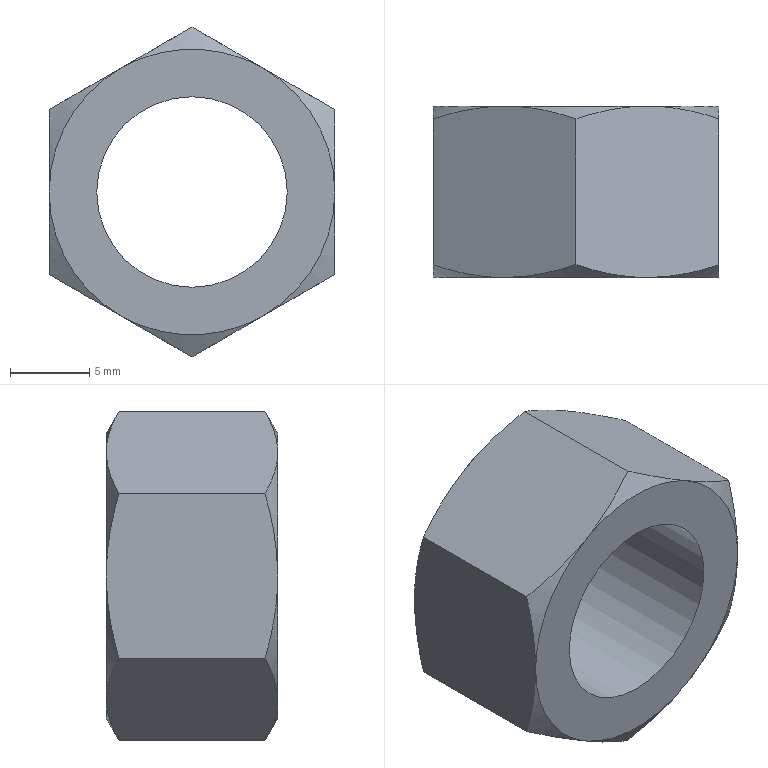Component | SolidWorks | GB_T6170-2000[Type1HexNutGradeAAndBM12]-1 | 1 solid | 22 faces | box 18 x 10.8 x 20.78 mm | volume 1796 mm3 | cone 12 | plane 8 | cylinder 2 | commonest cylinder face diameters 12 x2
build123d program:
from build123d import *

# Parameters (mm, degrees)
SKETCH1_R          = 6
BASE_EXTRUDE_DEPTH = 10.8
SKETCH2_OUTSIDE_W  = 89.934
SKETCH2_OUTSIDE_H  = 92.718
SKETCH2_OUTSIDE_R  = 9
CUT_EXTRUDE1_DEPTH = 18.483
CUT_EXTRUDE1_DRAFT = -60
SKETCH3_OUTSIDE_W  = 89.934
SKETCH3_OUTSIDE_H  = 92.718
SKETCH3_OUTSIDE_R  = 9
CUT_EXTRUDE2_DEPTH = 18.483
CUT_EXTRUDE2_DRAFT = -60


with BuildPart() as part:
    # Sketch1 → Base-Extrude (new body)
    with BuildSketch(Plane.XY):
        Polygon((0, 10.392), (-9, 5.196), (-9, -5.196), (0, -10.392), (9, -5.196), (9, 5.196), align=None)
        with Locations(Location((0, 0, 0), (0, 0, 180))):
            Circle(SKETCH1_R, mode=Mode.SUBTRACT)
    extrude(amount=BASE_EXTRUDE_DEPTH)


with BuildPart() as cut_extrude1_tool:
    # Sketch2 outside → Cut-Extrude1 (with draft: the straight prism first)
    with BuildSketch(Plane(origin=(0, 0, 0), x_dir=(-1, 0, 0), z_dir=(0, 0, -1))):
        Rectangle(SKETCH2_OUTSIDE_W, SKETCH2_OUTSIDE_H)
        Circle(SKETCH2_OUTSIDE_R, mode=Mode.SUBTRACT)
    extrude(amount=-CUT_EXTRUDE1_DEPTH)
    # Cut-Extrude1: the draft: its side faces are tilted about the plane it starts from
    cut_extrude1_sides = [cut_extrude1_tool.faces().sort_by_distance(p)[0] for p in [
        (0, -46.359, 9.241),
        (-44.967, 0, 9.241),
        (0, 46.359, 9.241),
        (44.967, 0, 9.241),
        (9, 0, 9.241),
    ]]
    draft(cut_extrude1_sides, Plane(origin=(0, 0, 0), x_dir=(-1, 0, 0), z_dir=(0, 0, -1)), CUT_EXTRUDE1_DRAFT)


with BuildPart() as part_1:
    add(part.part)

    # Cut-Extrude1: cut by cut_extrude1_tool
    add(cut_extrude1_tool.part, mode=Mode.SUBTRACT)


with BuildPart() as cut_extrude2_tool:
    # Sketch3 outside → Cut-Extrude2 (with draft: the straight prism first)
    with BuildSketch(Plane.XY.offset(10.8)):
        Rectangle(SKETCH3_OUTSIDE_W, SKETCH3_OUTSIDE_H)
        Circle(SKETCH3_OUTSIDE_R, mode=Mode.SUBTRACT)
    extrude(amount=-CUT_EXTRUDE2_DEPTH)
    # Cut-Extrude2: the draft: its side faces are tilted about the plane it starts from
    cut_extrude2_sides = [cut_extrude2_tool.faces().sort_by_distance(p)[0] for p in [
        (0, -46.359, 1.559),
        (44.967, 0, 1.559),
        (0, 46.359, 1.559),
        (-44.967, 0, 1.559),
        (-9, 0, 1.559),
    ]]
    draft(cut_extrude2_sides, Plane.XY.offset(10.8), CUT_EXTRUDE2_DRAFT)


with BuildPart() as part_2:
    add(part_1.part)

    # Cut-Extrude2: cut by cut_extrude2_tool
    add(cut_extrude2_tool.part, mode=Mode.SUBTRACT)


solid = part_2.part

# Placed as in the assembly
solid = solid.moved(Location((-380, -35.6, 90), (90, 0, 0)))
STEP:
#1=CARTESIAN_POINT('',(-15.197,-1.827,3.543));
#2=VERTEX_POINT('',#1);
#3=CARTESIAN_POINT('',(-14.724,-1.827,3.543));
#4=VERTEX_POINT('',#3);
#5=CARTESIAN_POINT('',(-14.961,-1.827,3.543));
#6=DIRECTION('',(0.,-1.,-0.));
#7=DIRECTION('',(1.,0.,0.));
#8=AXIS2_PLACEMENT_3D('',#5,#6,#7);
#9=CIRCLE('',#8,0.2362);
#10=EDGE_CURVE('',#2,#4,#9,.T.);
#11=ORIENTED_EDGE('',*,*,#10,.T.);
#12=CARTESIAN_POINT('',(-14.724,-1.402,3.543));
#13=VERTEX_POINT('',#12);
#14=CARTESIAN_POINT('',(-14.724,-1.827,3.543));
#15=DIRECTION('',(0.,1.,0.));
#16=VECTOR('',#15,39.37);
#17=LINE('',#14,#16);
#18=EDGE_CURVE('',#4,#13,#17,.T.);
#19=ORIENTED_EDGE('',*,*,#18,.T.);
#20=CARTESIAN_POINT('',(-15.197,-1.402,3.543));
#21=VERTEX_POINT('',#20);
#22=CARTESIAN_POINT('',(-14.961,-1.402,3.543));
#23=DIRECTION('',(0.,-1.,-0.));
#24=DIRECTION('',(1.,0.,0.));
#25=AXIS2_PLACEMENT_3D('',#22,#23,#24);
#26=CIRCLE('',#25,0.2362);
#27=EDGE_CURVE('',#21,#13,#26,.T.);
#28=ORIENTED_EDGE('',*,*,#27,.F.);
#29=CARTESIAN_POINT('',(-15.197,-1.827,3.543));
#30=DIRECTION('',(0.,1.,0.));
#31=VECTOR('',#30,39.37);
#32=LINE('',#29,#31);
#33=EDGE_CURVE('',#2,#21,#32,.T.);
#34=ORIENTED_EDGE('',*,*,#33,.F.);
#35=EDGE_LOOP('',(#11,#19,#28,#34));
#36=FACE_OUTER_BOUND('',#35,.T.);
#37=CARTESIAN_POINT('',(-14.961,-1.827,3.543));
#38=DIRECTION('',(0.,1.,0.));
#39=DIRECTION('',(-1.,0.,0.));
#40=AXIS2_PLACEMENT_3D('',#37,#38,#39);
#41=CYLINDRICAL_SURFACE('',#40,0.2362);
#42=ADVANCED_FACE('',(#36),#41,.F.);
#43=CARTESIAN_POINT('',(-14.606,-1.795,3.748));
#44=VERTEX_POINT('',#43);
#45=CARTESIAN_POINT('',(-14.783,-1.827,3.85));
#46=VERTEX_POINT('',#45);
#47=CARTESIAN_POINT('',(-14.606,-1.795,3.748));
#48=CARTESIAN_POINT('',(-14.635,-1.805,3.765));
#49=CARTESIAN_POINT('',(-14.664,-1.813,3.781));
#50=CARTESIAN_POINT('',(-14.723,-1.824,3.816));
#51=CARTESIAN_POINT('',(-14.753,-1.827,3.833));
#52=CARTESIAN_POINT('',(-14.783,-1.827,3.85));
#53=B_SPLINE_CURVE_WITH_KNOTS('',3,(#47,#48,#49,#50,#51,#52),.UNSPECIFIED.,.F.,.F.,(4,2,4),(0.00000024,0.002629,0.005258),.UNSPECIFIED.);
#54=EDGE_CURVE('',#44,#46,#53,.T.);
#55=ORIENTED_EDGE('',*,*,#54,.F.);
#56=CARTESIAN_POINT('',(-14.606,-1.433,3.748));
#57=VERTEX_POINT('',#56);
#58=CARTESIAN_POINT('',(-14.606,-1.827,3.748));
#59=DIRECTION('',(0.,1.,0.));
#60=VECTOR('',#59,39.37);
#61=LINE('',#58,#60);
#62=EDGE_CURVE('',#44,#57,#61,.T.);
#63=ORIENTED_EDGE('',*,*,#62,.T.);
#64=CARTESIAN_POINT('',(-14.783,-1.402,3.85));
#65=VERTEX_POINT('',#64);
#66=CARTESIAN_POINT('',(-14.783,-1.402,3.85));
#67=CARTESIAN_POINT('',(-14.768,-1.402,3.841));
#68=CARTESIAN_POINT('',(-14.753,-1.402,3.833));
#69=CARTESIAN_POINT('',(-14.723,-1.405,3.816));
#70=CARTESIAN_POINT('',(-14.709,-1.407,3.807));
#71=CARTESIAN_POINT('',(-14.664,-1.416,3.781));
#72=CARTESIAN_POINT('',(-14.635,-1.424,3.765));
#73=CARTESIAN_POINT('',(-14.606,-1.433,3.748));
#74=B_SPLINE_CURVE_WITH_KNOTS('',3,(#66,#67,#68,#69,#70,#71,#72,#73),.UNSPECIFIED.,.F.,.F.,(4,2,2,4),(0.005258,0.006567,0.007877,0.0105),.UNSPECIFIED.);
#75=EDGE_CURVE('',#65,#57,#74,.T.);
#76=ORIENTED_EDGE('',*,*,#75,.F.);
#77=CARTESIAN_POINT('',(-14.961,-1.433,3.952));
#78=VERTEX_POINT('',#77);
#79=CARTESIAN_POINT('',(-14.961,-1.433,3.952));
#80=CARTESIAN_POINT('',(-14.932,-1.424,3.936));
#81=CARTESIAN_POINT('',(-14.902,-1.416,3.919));
#82=CARTESIAN_POINT('',(-14.843,-1.405,3.885));
#83=CARTESIAN_POINT('',(-14.814,-1.402,3.868));
#84=CARTESIAN_POINT('',(-14.783,-1.402,3.85));
#85=B_SPLINE_CURVE_WITH_KNOTS('',3,(#79,#80,#81,#82,#83,#84),.UNSPECIFIED.,.F.,.F.,(4,2,4),(0.00000024,0.002629,0.005258),.UNSPECIFIED.);
#86=EDGE_CURVE('',#78,#65,#85,.T.);
#87=ORIENTED_EDGE('',*,*,#86,.F.);
#88=CARTESIAN_POINT('',(-14.961,-1.795,3.952));
#89=VERTEX_POINT('',#88);
#90=CARTESIAN_POINT('',(-14.961,-1.827,3.952));
#91=DIRECTION('',(0.,1.,0.));
#92=VECTOR('',#91,39.37);
#93=LINE('',#90,#92);
#94=EDGE_CURVE('',#89,#78,#93,.T.);
#95=ORIENTED_EDGE('',*,*,#94,.F.);
#96=CARTESIAN_POINT('',(-14.783,-1.827,3.85));
#97=CARTESIAN_POINT('',(-14.799,-1.827,3.859));
#98=CARTESIAN_POINT('',(-14.814,-1.826,3.868));
#99=CARTESIAN_POINT('',(-14.843,-1.823,3.885));
#100=CARTESIAN_POINT('',(-14.858,-1.821,3.893));
#101=CARTESIAN_POINT('',(-14.903,-1.813,3.919));
#102=CARTESIAN_POINT('',(-14.932,-1.805,3.936));
#103=CARTESIAN_POINT('',(-14.961,-1.795,3.952));
#104=B_SPLINE_CURVE_WITH_KNOTS('',3,(#96,#97,#98,#99,#100,#101,#102,#103),.UNSPECIFIED.,.F.,.F.,(4,2,2,4),(0.005258,0.006567,0.007877,0.0105),.UNSPECIFIED.);
#105=EDGE_CURVE('',#46,#89,#104,.T.);
#106=ORIENTED_EDGE('',*,*,#105,.F.);
#107=EDGE_LOOP('',(#55,#63,#76,#87,#95,#106));
#108=FACE_OUTER_BOUND('',#107,.T.);
#109=CARTESIAN_POINT('',(-14.606,-1.827,3.748));
#110=DIRECTION('',(-0.5,0.,-0.866));
#111=DIRECTION('',(0.866,0.,-0.5));
#112=AXIS2_PLACEMENT_3D('',#109,#110,#111);
#113=PLANE('',#112);
#114=ADVANCED_FACE('',(#108),#113,.F.);
#115=CARTESIAN_POINT('',(-15.138,-1.827,3.85));
#116=VERTEX_POINT('',#115);
#117=CARTESIAN_POINT('',(-14.961,-1.795,3.952));
#118=CARTESIAN_POINT('',(-14.99,-1.805,3.936));
#119=CARTESIAN_POINT('',(-15.019,-1.813,3.919));
#120=CARTESIAN_POINT('',(-15.078,-1.824,3.885));
#121=CARTESIAN_POINT('',(-15.108,-1.827,3.868));
#122=CARTESIAN_POINT('',(-15.138,-1.827,3.85));
#123=B_SPLINE_CURVE_WITH_KNOTS('',3,(#117,#118,#119,#120,#121,#122),.UNSPECIFIED.,.F.,.F.,(4,2,4),(0.00000024,0.002629,0.005258),.UNSPECIFIED.);
#124=EDGE_CURVE('',#89,#116,#123,.T.);
#125=ORIENTED_EDGE('',*,*,#124,.F.);
#126=ORIENTED_EDGE('',*,*,#94,.T.);
#127=CARTESIAN_POINT('',(-15.138,-1.402,3.85));
#128=VERTEX_POINT('',#127);
#129=CARTESIAN_POINT('',(-15.138,-1.402,3.85));
#130=CARTESIAN_POINT('',(-15.123,-1.402,3.859));
#131=CARTESIAN_POINT('',(-15.108,-1.402,3.868));
#132=CARTESIAN_POINT('',(-15.078,-1.405,3.885));
#133=CARTESIAN_POINT('',(-15.063,-1.407,3.893));
#134=CARTESIAN_POINT('',(-15.019,-1.416,3.919));
#135=CARTESIAN_POINT('',(-14.99,-1.424,3.936));
#136=CARTESIAN_POINT('',(-14.961,-1.433,3.952));
#137=B_SPLINE_CURVE_WITH_KNOTS('',3,(#129,#130,#131,#132,#133,#134,#135,#136),.UNSPECIFIED.,.F.,.F.,(4,2,2,4),(0.005258,0.006567,0.007877,0.0105),.UNSPECIFIED.);
#138=EDGE_CURVE('',#128,#78,#137,.T.);
#139=ORIENTED_EDGE('',*,*,#138,.F.);
#140=CARTESIAN_POINT('',(-15.315,-1.433,3.748));
#141=VERTEX_POINT('',#140);
#142=CARTESIAN_POINT('',(-15.315,-1.433,3.748));
#143=CARTESIAN_POINT('',(-15.286,-1.424,3.765));
#144=CARTESIAN_POINT('',(-15.257,-1.416,3.781));
#145=CARTESIAN_POINT('',(-15.198,-1.405,3.816));
#146=CARTESIAN_POINT('',(-15.168,-1.402,3.833));
#147=CARTESIAN_POINT('',(-15.138,-1.402,3.85));
#148=B_SPLINE_CURVE_WITH_KNOTS('',3,(#142,#143,#144,#145,#146,#147),.UNSPECIFIED.,.F.,.F.,(4,2,4),(0.00000024,0.002629,0.005258),.UNSPECIFIED.);
#149=EDGE_CURVE('',#141,#128,#148,.T.);
#150=ORIENTED_EDGE('',*,*,#149,.F.);
#151=CARTESIAN_POINT('',(-15.315,-1.795,3.748));
#152=VERTEX_POINT('',#151);
#153=CARTESIAN_POINT('',(-15.315,-1.827,3.748));
#154=DIRECTION('',(0.,1.,0.));
#155=VECTOR('',#154,39.37);
#156=LINE('',#153,#155);
#157=EDGE_CURVE('',#152,#141,#156,.T.);
#158=ORIENTED_EDGE('',*,*,#157,.F.);
#159=CARTESIAN_POINT('',(-15.138,-1.827,3.85));
#160=CARTESIAN_POINT('',(-15.153,-1.827,3.841));
#161=CARTESIAN_POINT('',(-15.168,-1.826,3.833));
#162=CARTESIAN_POINT('',(-15.198,-1.823,3.816));
#163=CARTESIAN_POINT('',(-15.213,-1.821,3.807));
#164=CARTESIAN_POINT('',(-15.257,-1.813,3.781));
#165=CARTESIAN_POINT('',(-15.286,-1.805,3.765));
#166=CARTESIAN_POINT('',(-15.315,-1.795,3.748));
#167=B_SPLINE_CURVE_WITH_KNOTS('',3,(#159,#160,#161,#162,#163,#164,#165,#166),.UNSPECIFIED.,.F.,.F.,(4,2,2,4),(0.005258,0.006567,0.007877,0.0105),.UNSPECIFIED.);
#168=EDGE_CURVE('',#116,#152,#167,.T.);
#169=ORIENTED_EDGE('',*,*,#168,.F.);
#170=EDGE_LOOP('',(#125,#126,#139,#150,#158,#169));
#171=FACE_OUTER_BOUND('',#170,.T.);
#172=CARTESIAN_POINT('',(-14.961,-1.827,3.952));
#173=DIRECTION('',(0.5,0.,-0.866));
#174=DIRECTION('',(0.866,-0.,0.5));
#175=AXIS2_PLACEMENT_3D('',#172,#173,#174);
#176=PLANE('',#175);
#177=ADVANCED_FACE('',(#171),#176,.F.);
#178=CARTESIAN_POINT('',(-15.315,-1.827,3.543));
#179=VERTEX_POINT('',#178);
#180=CARTESIAN_POINT('',(-15.315,-1.795,3.748));
#181=CARTESIAN_POINT('',(-15.315,-1.805,3.715));
#182=CARTESIAN_POINT('',(-15.315,-1.813,3.681));
#183=CARTESIAN_POINT('',(-15.315,-1.821,3.63));
#184=CARTESIAN_POINT('',(-15.315,-1.823,3.613));
#185=CARTESIAN_POINT('',(-15.315,-1.826,3.578));
#186=CARTESIAN_POINT('',(-15.315,-1.827,3.561));
#187=CARTESIAN_POINT('',(-15.315,-1.827,3.543));
#188=B_SPLINE_CURVE_WITH_KNOTS('',3,(#180,#181,#182,#183,#184,#185,#186,#187),.UNSPECIFIED.,.F.,.F.,(4,2,2,4),(0.02958,0.03221,0.03352,0.03484),.UNSPECIFIED.);
#189=EDGE_CURVE('',#152,#179,#188,.T.);
#190=ORIENTED_EDGE('',*,*,#189,.F.);
#191=ORIENTED_EDGE('',*,*,#157,.T.);
#192=CARTESIAN_POINT('',(-15.315,-1.402,3.543));
#193=VERTEX_POINT('',#192);
#194=CARTESIAN_POINT('',(-15.315,-1.402,3.543));
#195=CARTESIAN_POINT('',(-15.315,-1.402,3.561));
#196=CARTESIAN_POINT('',(-15.315,-1.402,3.578));
#197=CARTESIAN_POINT('',(-15.315,-1.405,3.613));
#198=CARTESIAN_POINT('',(-15.315,-1.407,3.63));
#199=CARTESIAN_POINT('',(-15.315,-1.416,3.681));
#200=CARTESIAN_POINT('',(-15.315,-1.424,3.715));
#201=CARTESIAN_POINT('',(-15.315,-1.433,3.748));
#202=B_SPLINE_CURVE_WITH_KNOTS('',3,(#194,#195,#196,#197,#198,#199,#200,#201),.UNSPECIFIED.,.F.,.F.,(4,2,2,4),(0.01478,0.01609,0.01741,0.02004),.UNSPECIFIED.);
#203=EDGE_CURVE('',#193,#141,#202,.T.);
#204=ORIENTED_EDGE('',*,*,#203,.F.);
#205=CARTESIAN_POINT('',(-15.315,-1.433,3.339));
#206=VERTEX_POINT('',#205);
#207=CARTESIAN_POINT('',(-15.315,-1.433,3.339));
#208=CARTESIAN_POINT('',(-15.315,-1.424,3.372));
#209=CARTESIAN_POINT('',(-15.315,-1.416,3.406));
#210=CARTESIAN_POINT('',(-15.315,-1.405,3.474));
#211=CARTESIAN_POINT('',(-15.315,-1.402,3.509));
#212=CARTESIAN_POINT('',(-15.315,-1.402,3.543));
#213=B_SPLINE_CURVE_WITH_KNOTS('',3,(#207,#208,#209,#210,#211,#212),.UNSPECIFIED.,.F.,.F.,(4,2,4),(0.009518,0.01215,0.01478),.UNSPECIFIED.);
#214=EDGE_CURVE('',#206,#193,#213,.T.);
#215=ORIENTED_EDGE('',*,*,#214,.F.);
#216=CARTESIAN_POINT('',(-15.315,-1.795,3.339));
#217=VERTEX_POINT('',#216);
#218=CARTESIAN_POINT('',(-15.315,-1.827,3.339));
#219=DIRECTION('',(0.,1.,0.));
#220=VECTOR('',#219,39.37);
#221=LINE('',#218,#220);
#222=EDGE_CURVE('',#217,#206,#221,.T.);
#223=ORIENTED_EDGE('',*,*,#222,.F.);
#224=CARTESIAN_POINT('',(-15.315,-1.827,3.543));
#225=CARTESIAN_POINT('',(-15.315,-1.827,3.509));
#226=CARTESIAN_POINT('',(-15.315,-1.824,3.474));
#227=CARTESIAN_POINT('',(-15.315,-1.813,3.406));
#228=CARTESIAN_POINT('',(-15.315,-1.805,3.372));
#229=CARTESIAN_POINT('',(-15.315,-1.795,3.339));
#230=B_SPLINE_CURVE_WITH_KNOTS('',3,(#224,#225,#226,#227,#228,#229),.UNSPECIFIED.,.F.,.F.,(4,2,4),(0.03484,0.03747,0.0401),.UNSPECIFIED.);
#231=EDGE_CURVE('',#179,#217,#230,.T.);
#232=ORIENTED_EDGE('',*,*,#231,.F.);
#233=EDGE_LOOP('',(#190,#191,#204,#215,#223,#232));
#234=FACE_OUTER_BOUND('',#233,.T.);
#235=CARTESIAN_POINT('',(-15.315,-1.827,3.748));
#236=DIRECTION('',(1.,-0.,0.));
#237=DIRECTION('',(-0.,-0.,1.));
#238=AXIS2_PLACEMENT_3D('',#235,#236,#237);
#239=PLANE('',#238);
#240=ADVANCED_FACE('',(#234),#239,.F.);
#241=CARTESIAN_POINT('',(-15.138,-1.827,3.236));
#242=VERTEX_POINT('',#241);
#243=CARTESIAN_POINT('',(-15.315,-1.795,3.339));
#244=CARTESIAN_POINT('',(-15.286,-1.805,3.322));
#245=CARTESIAN_POINT('',(-15.257,-1.813,3.305));
#246=CARTESIAN_POINT('',(-15.198,-1.824,3.271));
#247=CARTESIAN_POINT('',(-15.168,-1.827,3.254));
#248=CARTESIAN_POINT('',(-15.138,-1.827,3.236));
#249=B_SPLINE_CURVE_WITH_KNOTS('',3,(#243,#244,#245,#246,#247,#248),.UNSPECIFIED.,.F.,.F.,(4,2,4),(0.00000024,0.002629,0.005258),.UNSPECIFIED.);
#250=EDGE_CURVE('',#217,#242,#249,.T.);
#251=ORIENTED_EDGE('',*,*,#250,.F.);
#252=ORIENTED_EDGE('',*,*,#222,.T.);
#253=CARTESIAN_POINT('',(-15.138,-1.402,3.236));
#254=VERTEX_POINT('',#253);
#255=CARTESIAN_POINT('',(-15.138,-1.402,3.236));
#256=CARTESIAN_POINT('',(-15.153,-1.402,3.245));
#257=CARTESIAN_POINT('',(-15.168,-1.402,3.254));
#258=CARTESIAN_POINT('',(-15.198,-1.405,3.271));
#259=CARTESIAN_POINT('',(-15.213,-1.407,3.28));
#260=CARTESIAN_POINT('',(-15.257,-1.416,3.305));
#261=CARTESIAN_POINT('',(-15.286,-1.424,3.322));
#262=CARTESIAN_POINT('',(-15.315,-1.433,3.339));
#263=B_SPLINE_CURVE_WITH_KNOTS('',3,(#255,#256,#257,#258,#259,#260,#261,#262),.UNSPECIFIED.,.F.,.F.,(4,2,2,4),(0.005258,0.006567,0.007877,0.0105),.UNSPECIFIED.);
#264=EDGE_CURVE('',#254,#206,#263,.T.);
#265=ORIENTED_EDGE('',*,*,#264,.F.);
#266=CARTESIAN_POINT('',(-14.961,-1.433,3.134));
#267=VERTEX_POINT('',#266);
#268=CARTESIAN_POINT('',(-14.961,-1.433,3.134));
#269=CARTESIAN_POINT('',(-14.99,-1.424,3.151));
#270=CARTESIAN_POINT('',(-15.019,-1.416,3.168));
#271=CARTESIAN_POINT('',(-15.078,-1.405,3.202));
#272=CARTESIAN_POINT('',(-15.108,-1.402,3.219));
#273=CARTESIAN_POINT('',(-15.138,-1.402,3.236));
#274=B_SPLINE_CURVE_WITH_KNOTS('',3,(#268,#269,#270,#271,#272,#273),.UNSPECIFIED.,.F.,.F.,(4,2,4),(0.00000024,0.002629,0.005258),.UNSPECIFIED.);
#275=EDGE_CURVE('',#267,#254,#274,.T.);
#276=ORIENTED_EDGE('',*,*,#275,.F.);
#277=CARTESIAN_POINT('',(-14.961,-1.795,3.134));
#278=VERTEX_POINT('',#277);
#279=CARTESIAN_POINT('',(-14.961,-1.827,3.134));
#280=DIRECTION('',(0.,1.,0.));
#281=VECTOR('',#280,39.37);
#282=LINE('',#279,#281);
#283=EDGE_CURVE('',#278,#267,#282,.T.);
#284=ORIENTED_EDGE('',*,*,#283,.F.);
#285=CARTESIAN_POINT('',(-15.138,-1.827,3.236));
#286=CARTESIAN_POINT('',(-15.123,-1.827,3.228));
#287=CARTESIAN_POINT('',(-15.108,-1.826,3.219));
#288=CARTESIAN_POINT('',(-15.078,-1.823,3.202));
#289=CARTESIAN_POINT('',(-15.063,-1.821,3.193));
#290=CARTESIAN_POINT('',(-15.019,-1.813,3.168));
#291=CARTESIAN_POINT('',(-14.99,-1.805,3.151));
#292=CARTESIAN_POINT('',(-14.961,-1.795,3.134));
#293=B_SPLINE_CURVE_WITH_KNOTS('',3,(#285,#286,#287,#288,#289,#290,#291,#292),.UNSPECIFIED.,.F.,.F.,(4,2,2,4),(0.005258,0.006567,0.007877,0.0105),.UNSPECIFIED.);
#294=EDGE_CURVE('',#242,#278,#293,.T.);
#295=ORIENTED_EDGE('',*,*,#294,.F.);
#296=EDGE_LOOP('',(#251,#252,#265,#276,#284,#295));
#297=FACE_OUTER_BOUND('',#296,.T.);
#298=CARTESIAN_POINT('',(-15.315,-1.827,3.339));
#299=DIRECTION('',(0.5,-0.,0.866));
#300=DIRECTION('',(-0.866,-0.,0.5));
#301=AXIS2_PLACEMENT_3D('',#298,#299,#300);
#302=PLANE('',#301);
#303=ADVANCED_FACE('',(#297),#302,.F.);
#304=CARTESIAN_POINT('',(-14.783,-1.827,3.236));
#305=VERTEX_POINT('',#304);
#306=CARTESIAN_POINT('',(-14.961,-1.795,3.134));
#307=CARTESIAN_POINT('',(-14.932,-1.805,3.151));
#308=CARTESIAN_POINT('',(-14.902,-1.813,3.168));
#309=CARTESIAN_POINT('',(-14.843,-1.824,3.202));
#310=CARTESIAN_POINT('',(-14.814,-1.827,3.219));
#311=CARTESIAN_POINT('',(-14.783,-1.827,3.236));
#312=B_SPLINE_CURVE_WITH_KNOTS('',3,(#306,#307,#308,#309,#310,#311),.UNSPECIFIED.,.F.,.F.,(4,2,4),(0.00000024,0.002629,0.005258),.UNSPECIFIED.);
#313=EDGE_CURVE('',#278,#305,#312,.T.);
#314=ORIENTED_EDGE('',*,*,#313,.F.);
#315=ORIENTED_EDGE('',*,*,#283,.T.);
#316=CARTESIAN_POINT('',(-14.783,-1.402,3.236));
#317=VERTEX_POINT('',#316);
#318=CARTESIAN_POINT('',(-14.783,-1.402,3.236));
#319=CARTESIAN_POINT('',(-14.799,-1.402,3.228));
#320=CARTESIAN_POINT('',(-14.814,-1.402,3.219));
#321=CARTESIAN_POINT('',(-14.843,-1.405,3.202));
#322=CARTESIAN_POINT('',(-14.858,-1.407,3.193));
#323=CARTESIAN_POINT('',(-14.903,-1.416,3.168));
#324=CARTESIAN_POINT('',(-14.932,-1.424,3.151));
#325=CARTESIAN_POINT('',(-14.961,-1.433,3.134));
#326=B_SPLINE_CURVE_WITH_KNOTS('',3,(#318,#319,#320,#321,#322,#323,#324,#325),.UNSPECIFIED.,.F.,.F.,(4,2,2,4),(0.005258,0.006567,0.007877,0.0105),.UNSPECIFIED.);
#327=EDGE_CURVE('',#317,#267,#326,.T.);
#328=ORIENTED_EDGE('',*,*,#327,.F.);
#329=CARTESIAN_POINT('',(-14.606,-1.433,3.339));
#330=VERTEX_POINT('',#329);
#331=CARTESIAN_POINT('',(-14.606,-1.433,3.339));
#332=CARTESIAN_POINT('',(-14.635,-1.424,3.322));
#333=CARTESIAN_POINT('',(-14.664,-1.416,3.305));
#334=CARTESIAN_POINT('',(-14.723,-1.405,3.271));
#335=CARTESIAN_POINT('',(-14.753,-1.402,3.254));
#336=CARTESIAN_POINT('',(-14.783,-1.402,3.236));
#337=B_SPLINE_CURVE_WITH_KNOTS('',3,(#331,#332,#333,#334,#335,#336),.UNSPECIFIED.,.F.,.F.,(4,2,4),(0.00000024,0.002629,0.005258),.UNSPECIFIED.);
#338=EDGE_CURVE('',#330,#317,#337,.T.);
#339=ORIENTED_EDGE('',*,*,#338,.F.);
#340=CARTESIAN_POINT('',(-14.606,-1.795,3.339));
#341=VERTEX_POINT('',#340);
#342=CARTESIAN_POINT('',(-14.606,-1.827,3.339));
#343=DIRECTION('',(0.,1.,0.));
#344=VECTOR('',#343,39.37);
#345=LINE('',#342,#344);
#346=EDGE_CURVE('',#341,#330,#345,.T.);
#347=ORIENTED_EDGE('',*,*,#346,.F.);
#348=CARTESIAN_POINT('',(-14.783,-1.827,3.236));
#349=CARTESIAN_POINT('',(-14.768,-1.827,3.245));
#350=CARTESIAN_POINT('',(-14.753,-1.826,3.254));
#351=CARTESIAN_POINT('',(-14.723,-1.823,3.271));
#352=CARTESIAN_POINT('',(-14.709,-1.821,3.28));
#353=CARTESIAN_POINT('',(-14.664,-1.813,3.305));
#354=CARTESIAN_POINT('',(-14.635,-1.805,3.322));
#355=CARTESIAN_POINT('',(-14.606,-1.795,3.339));
#356=B_SPLINE_CURVE_WITH_KNOTS('',3,(#348,#349,#350,#351,#352,#353,#354,#355),.UNSPECIFIED.,.F.,.F.,(4,2,2,4),(0.005258,0.006567,0.007877,0.0105),.UNSPECIFIED.);
#357=EDGE_CURVE('',#305,#341,#356,.T.);
#358=ORIENTED_EDGE('',*,*,#357,.F.);
#359=EDGE_LOOP('',(#314,#315,#328,#339,#347,#358));
#360=FACE_OUTER_BOUND('',#359,.T.);
#361=CARTESIAN_POINT('',(-14.961,-1.827,3.134));
#362=DIRECTION('',(-0.5,-0.,0.866));
#363=DIRECTION('',(-0.866,0.,-0.5));
#364=AXIS2_PLACEMENT_3D('',#361,#362,#363);
#365=PLANE('',#364);
#366=ADVANCED_FACE('',(#360),#365,.F.);
#367=CARTESIAN_POINT('',(-14.606,-1.827,3.543));
#368=VERTEX_POINT('',#367);
#369=CARTESIAN_POINT('',(-14.606,-1.795,3.339));
#370=CARTESIAN_POINT('',(-14.606,-1.805,3.372));
#371=CARTESIAN_POINT('',(-14.606,-1.813,3.406));
#372=CARTESIAN_POINT('',(-14.606,-1.824,3.474));
#373=CARTESIAN_POINT('',(-14.606,-1.827,3.509));
#374=CARTESIAN_POINT('',(-14.606,-1.827,3.543));
#375=B_SPLINE_CURVE_WITH_KNOTS('',3,(#369,#370,#371,#372,#373,#374),.UNSPECIFIED.,.F.,.F.,(4,2,4),(0.009518,0.01215,0.01478),.UNSPECIFIED.);
#376=EDGE_CURVE('',#341,#368,#375,.T.);
#377=ORIENTED_EDGE('',*,*,#376,.F.);
#378=ORIENTED_EDGE('',*,*,#346,.T.);
#379=CARTESIAN_POINT('',(-14.606,-1.402,3.543));
#380=VERTEX_POINT('',#379);
#381=CARTESIAN_POINT('',(-14.606,-1.402,3.543));
#382=CARTESIAN_POINT('',(-14.606,-1.402,3.509));
#383=CARTESIAN_POINT('',(-14.606,-1.405,3.474));
#384=CARTESIAN_POINT('',(-14.606,-1.416,3.406));
#385=CARTESIAN_POINT('',(-14.606,-1.424,3.372));
#386=CARTESIAN_POINT('',(-14.606,-1.433,3.339));
#387=B_SPLINE_CURVE_WITH_KNOTS('',3,(#381,#382,#383,#384,#385,#386),.UNSPECIFIED.,.F.,.F.,(4,2,4),(0.03484,0.03747,0.0401),.UNSPECIFIED.);
#388=EDGE_CURVE('',#380,#330,#387,.T.);
#389=ORIENTED_EDGE('',*,*,#388,.F.);
#390=CARTESIAN_POINT('',(-14.606,-1.433,3.748));
#391=CARTESIAN_POINT('',(-14.606,-1.424,3.715));
#392=CARTESIAN_POINT('',(-14.606,-1.416,3.681));
#393=CARTESIAN_POINT('',(-14.606,-1.407,3.63));
#394=CARTESIAN_POINT('',(-14.606,-1.405,3.613));
#395=CARTESIAN_POINT('',(-14.606,-1.402,3.578));
#396=CARTESIAN_POINT('',(-14.606,-1.402,3.561));
#397=CARTESIAN_POINT('',(-14.606,-1.402,3.543));
#398=B_SPLINE_CURVE_WITH_KNOTS('',3,(#390,#391,#392,#393,#394,#395,#396,#397),.UNSPECIFIED.,.F.,.F.,(4,2,2,4),(0.02958,0.03221,0.03352,0.03484),.UNSPECIFIED.);
#399=EDGE_CURVE('',#57,#380,#398,.T.);
#400=ORIENTED_EDGE('',*,*,#399,.F.);
#401=ORIENTED_EDGE('',*,*,#62,.F.);
#402=CARTESIAN_POINT('',(-14.606,-1.827,3.543));
#403=CARTESIAN_POINT('',(-14.606,-1.827,3.561));
#404=CARTESIAN_POINT('',(-14.606,-1.826,3.578));
#405=CARTESIAN_POINT('',(-14.606,-1.823,3.613));
#406=CARTESIAN_POINT('',(-14.606,-1.821,3.63));
#407=CARTESIAN_POINT('',(-14.606,-1.813,3.681));
#408=CARTESIAN_POINT('',(-14.606,-1.805,3.715));
#409=CARTESIAN_POINT('',(-14.606,-1.795,3.748));
#410=B_SPLINE_CURVE_WITH_KNOTS('',3,(#402,#403,#404,#405,#406,#407,#408,#409),.UNSPECIFIED.,.F.,.F.,(4,2,2,4),(0.01478,0.01609,0.01741,0.02004),.UNSPECIFIED.);
#411=EDGE_CURVE('',#368,#44,#410,.T.);
#412=ORIENTED_EDGE('',*,*,#411,.F.);
#413=EDGE_LOOP('',(#377,#378,#389,#400,#401,#412));
#414=FACE_OUTER_BOUND('',#413,.T.);
#415=CARTESIAN_POINT('',(-14.606,-1.827,3.339));
#416=DIRECTION('',(-1.,0.,-0.));
#417=DIRECTION('',(0.,0.,-1.));
#418=AXIS2_PLACEMENT_3D('',#415,#416,#417);
#419=PLANE('',#418);
#420=ADVANCED_FACE('',(#414),#419,.F.);
#421=ORIENTED_EDGE('',*,*,#10,.F.);
#422=CARTESIAN_POINT('',(-14.961,-1.827,3.543));
#423=DIRECTION('',(0.,-1.,-0.));
#424=DIRECTION('',(1.,0.,0.));
#425=AXIS2_PLACEMENT_3D('',#422,#423,#424);
#426=CIRCLE('',#425,0.2362);
#427=EDGE_CURVE('',#4,#2,#426,.T.);
#428=ORIENTED_EDGE('',*,*,#427,.F.);
#429=EDGE_LOOP('',(#421,#428));
#430=FACE_BOUND('',#429,.T.);
#431=CARTESIAN_POINT('',(-14.961,-1.827,3.543));
#432=DIRECTION('',(0.,-1.,-0.));
#433=DIRECTION('',(1.,0.,0.));
#434=AXIS2_PLACEMENT_3D('',#431,#432,#433);
#435=CIRCLE('',#434,0.3543);
#436=EDGE_CURVE('',#305,#368,#435,.T.);
#437=ORIENTED_EDGE('',*,*,#436,.T.);
#438=CARTESIAN_POINT('',(-14.961,-1.827,3.543));
#439=DIRECTION('',(0.,-1.,-0.));
#440=DIRECTION('',(1.,0.,0.));
#441=AXIS2_PLACEMENT_3D('',#438,#439,#440);
#442=CIRCLE('',#441,0.3543);
#443=EDGE_CURVE('',#368,#46,#442,.T.);
#444=ORIENTED_EDGE('',*,*,#443,.T.);
#445=CARTESIAN_POINT('',(-14.961,-1.827,3.543));
#446=DIRECTION('',(0.,-1.,-0.));
#447=DIRECTION('',(1.,0.,0.));
#448=AXIS2_PLACEMENT_3D('',#445,#446,#447);
#449=CIRCLE('',#448,0.3543);
#450=EDGE_CURVE('',#46,#116,#449,.T.);
#451=ORIENTED_EDGE('',*,*,#450,.T.);
#452=CARTESIAN_POINT('',(-14.961,-1.827,3.543));
#453=DIRECTION('',(0.,-1.,-0.));
#454=DIRECTION('',(1.,0.,0.));
#455=AXIS2_PLACEMENT_3D('',#452,#453,#454);
#456=CIRCLE('',#455,0.3543);
#457=EDGE_CURVE('',#116,#179,#456,.T.);
#458=ORIENTED_EDGE('',*,*,#457,.T.);
#459=CARTESIAN_POINT('',(-14.961,-1.827,3.543));
#460=DIRECTION('',(0.,-1.,-0.));
#461=DIRECTION('',(1.,0.,0.));
#462=AXIS2_PLACEMENT_3D('',#459,#460,#461);
#463=CIRCLE('',#462,0.3543);
#464=EDGE_CURVE('',#179,#242,#463,.T.);
#465=ORIENTED_EDGE('',*,*,#464,.T.);
#466=CARTESIAN_POINT('',(-14.961,-1.827,3.543));
#467=DIRECTION('',(0.,-1.,-0.));
#468=DIRECTION('',(1.,0.,0.));
#469=AXIS2_PLACEMENT_3D('',#466,#467,#468);
#470=CIRCLE('',#469,0.3543);
#471=EDGE_CURVE('',#242,#305,#470,.T.);
#472=ORIENTED_EDGE('',*,*,#471,.T.);
#473=EDGE_LOOP('',(#437,#444,#451,#458,#465,#472));
#474=FACE_OUTER_BOUND('',#473,.T.);
#475=CARTESIAN_POINT('',(-15.315,-1.827,4.157));
#476=DIRECTION('',(0.,-1.,-0.));
#477=DIRECTION('',(1.,0.,0.));
#478=AXIS2_PLACEMENT_3D('',#475,#476,#477);
#479=PLANE('',#478);
#480=ADVANCED_FACE('',(#430,#474),#479,.T.);
#481=ORIENTED_EDGE('',*,*,#27,.T.);
#482=CARTESIAN_POINT('',(-14.961,-1.402,3.543));
#483=DIRECTION('',(0.,-1.,-0.));
#484=DIRECTION('',(1.,0.,0.));
#485=AXIS2_PLACEMENT_3D('',#482,#483,#484);
#486=CIRCLE('',#485,0.2362);
#487=EDGE_CURVE('',#13,#21,#486,.T.);
#488=ORIENTED_EDGE('',*,*,#487,.T.);
#489=EDGE_LOOP('',(#481,#488));
#490=FACE_BOUND('',#489,.T.);
#491=CARTESIAN_POINT('',(-14.961,-1.402,3.543));
#492=DIRECTION('',(0.,1.,0.));
#493=DIRECTION('',(-1.,0.,0.));
#494=AXIS2_PLACEMENT_3D('',#491,#492,#493);
#495=CIRCLE('',#494,0.3543);
#496=EDGE_CURVE('',#65,#380,#495,.T.);
#497=ORIENTED_EDGE('',*,*,#496,.T.);
#498=CARTESIAN_POINT('',(-14.961,-1.402,3.543));
#499=DIRECTION('',(0.,1.,0.));
#500=DIRECTION('',(-1.,0.,0.));
#501=AXIS2_PLACEMENT_3D('',#498,#499,#500);
#502=CIRCLE('',#501,0.3543);
#503=EDGE_CURVE('',#380,#317,#502,.T.);
#504=ORIENTED_EDGE('',*,*,#503,.T.);
#505=CARTESIAN_POINT('',(-14.961,-1.402,3.543));
#506=DIRECTION('',(0.,1.,0.));
#507=DIRECTION('',(-1.,0.,0.));
#508=AXIS2_PLACEMENT_3D('',#505,#506,#507);
#509=CIRCLE('',#508,0.3543);
#510=EDGE_CURVE('',#317,#254,#509,.T.);
#511=ORIENTED_EDGE('',*,*,#510,.T.);
#512=CARTESIAN_POINT('',(-14.961,-1.402,3.543));
#513=DIRECTION('',(0.,1.,0.));
#514=DIRECTION('',(-1.,0.,0.));
#515=AXIS2_PLACEMENT_3D('',#512,#513,#514);
#516=CIRCLE('',#515,0.3543);
#517=EDGE_CURVE('',#254,#193,#516,.T.);
#518=ORIENTED_EDGE('',*,*,#517,.T.);
#519=CARTESIAN_POINT('',(-14.961,-1.402,3.543));
#520=DIRECTION('',(0.,1.,0.));
#521=DIRECTION('',(-1.,0.,0.));
#522=AXIS2_PLACEMENT_3D('',#519,#520,#521);
#523=CIRCLE('',#522,0.3543);
#524=EDGE_CURVE('',#193,#128,#523,.T.);
#525=ORIENTED_EDGE('',*,*,#524,.T.);
#526=CARTESIAN_POINT('',(-14.961,-1.402,3.543));
#527=DIRECTION('',(0.,1.,0.));
#528=DIRECTION('',(-1.,0.,0.));
#529=AXIS2_PLACEMENT_3D('',#526,#527,#528);
#530=CIRCLE('',#529,0.3543);
#531=EDGE_CURVE('',#128,#65,#530,.T.);
#532=ORIENTED_EDGE('',*,*,#531,.T.);
#533=EDGE_LOOP('',(#497,#504,#511,#518,#525,#532));
#534=FACE_OUTER_BOUND('',#533,.T.);
#535=CARTESIAN_POINT('',(-15.315,-1.402,4.157));
#536=DIRECTION('',(0.,-1.,-0.));
#537=DIRECTION('',(1.,0.,0.));
#538=AXIS2_PLACEMENT_3D('',#535,#536,#537);
#539=PLANE('',#538);
#540=ADVANCED_FACE('',(#490,#534),#539,.F.);
#541=ORIENTED_EDGE('',*,*,#18,.F.);
#542=ORIENTED_EDGE('',*,*,#427,.T.);
#543=ORIENTED_EDGE('',*,*,#33,.T.);
#544=ORIENTED_EDGE('',*,*,#487,.F.);
#545=EDGE_LOOP('',(#541,#542,#543,#544));
#546=FACE_OUTER_BOUND('',#545,.T.);
#547=CARTESIAN_POINT('',(-14.961,-1.827,3.543));
#548=DIRECTION('',(0.,1.,0.));
#549=DIRECTION('',(-1.,0.,0.));
#550=AXIS2_PLACEMENT_3D('',#547,#548,#549);
#551=CYLINDRICAL_SURFACE('',#550,0.2362);
#552=ADVANCED_FACE('',(#546),#551,.F.);
#553=ORIENTED_EDGE('',*,*,#338,.T.);
#554=ORIENTED_EDGE('',*,*,#503,.F.);
#555=ORIENTED_EDGE('',*,*,#388,.T.);
#556=EDGE_LOOP('',(#553,#554,#555));
#557=FACE_OUTER_BOUND('',#556,.T.);
#558=CARTESIAN_POINT('',(-14.961,-1.402,3.543));
#559=DIRECTION('',(0.,-1.,-0.));
#560=DIRECTION('',(-1.,0.,0.));
#561=AXIS2_PLACEMENT_3D('',#558,#559,#560);
#562=CONICAL_SURFACE('',#561,0.3543,1.047);
#563=ADVANCED_FACE('',(#557),#562,.T.);
#564=ORIENTED_EDGE('',*,*,#75,.T.);
#565=ORIENTED_EDGE('',*,*,#399,.T.);
#566=ORIENTED_EDGE('',*,*,#496,.F.);
#567=EDGE_LOOP('',(#564,#565,#566));
#568=FACE_OUTER_BOUND('',#567,.T.);
#569=CARTESIAN_POINT('',(-14.961,-1.402,3.543));
#570=DIRECTION('',(0.,-1.,-0.));
#571=DIRECTION('',(-1.,0.,0.));
#572=AXIS2_PLACEMENT_3D('',#569,#570,#571);
#573=CONICAL_SURFACE('',#572,0.3543,1.047);
#574=ADVANCED_FACE('',(#568),#573,.T.);
#575=ORIENTED_EDGE('',*,*,#275,.T.);
#576=ORIENTED_EDGE('',*,*,#510,.F.);
#577=ORIENTED_EDGE('',*,*,#327,.T.);
#578=EDGE_LOOP('',(#575,#576,#577));
#579=FACE_OUTER_BOUND('',#578,.T.);
#580=CARTESIAN_POINT('',(-14.961,-1.402,3.543));
#581=DIRECTION('',(0.,-1.,-0.));
#582=DIRECTION('',(-1.,0.,0.));
#583=AXIS2_PLACEMENT_3D('',#580,#581,#582);
#584=CONICAL_SURFACE('',#583,0.3543,1.047);
#585=ADVANCED_FACE('',(#579),#584,.T.);
#586=ORIENTED_EDGE('',*,*,#214,.T.);
#587=ORIENTED_EDGE('',*,*,#517,.F.);
#588=ORIENTED_EDGE('',*,*,#264,.T.);
#589=EDGE_LOOP('',(#586,#587,#588));
#590=FACE_OUTER_BOUND('',#589,.T.);
#591=CARTESIAN_POINT('',(-14.961,-1.402,3.543));
#592=DIRECTION('',(0.,-1.,-0.));
#593=DIRECTION('',(-1.,0.,0.));
#594=AXIS2_PLACEMENT_3D('',#591,#592,#593);
#595=CONICAL_SURFACE('',#594,0.3543,1.047);
#596=ADVANCED_FACE('',(#590),#595,.T.);
#597=ORIENTED_EDGE('',*,*,#203,.T.);
#598=ORIENTED_EDGE('',*,*,#149,.T.);
#599=ORIENTED_EDGE('',*,*,#524,.F.);
#600=EDGE_LOOP('',(#597,#598,#599));
#601=FACE_OUTER_BOUND('',#600,.T.);
#602=CARTESIAN_POINT('',(-14.961,-1.402,3.543));
#603=DIRECTION('',(0.,-1.,-0.));
#604=DIRECTION('',(-1.,0.,0.));
#605=AXIS2_PLACEMENT_3D('',#602,#603,#604);
#606=CONICAL_SURFACE('',#605,0.3543,1.047);
#607=ADVANCED_FACE('',(#601),#606,.T.);
#608=ORIENTED_EDGE('',*,*,#138,.T.);
#609=ORIENTED_EDGE('',*,*,#86,.T.);
#610=ORIENTED_EDGE('',*,*,#531,.F.);
#611=EDGE_LOOP('',(#608,#609,#610));
#612=FACE_OUTER_BOUND('',#611,.T.);
#613=CARTESIAN_POINT('',(-14.961,-1.402,3.543));
#614=DIRECTION('',(0.,-1.,-0.));
#615=DIRECTION('',(-1.,0.,0.));
#616=AXIS2_PLACEMENT_3D('',#613,#614,#615);
#617=CONICAL_SURFACE('',#616,0.3543,1.047);
#618=ADVANCED_FACE('',(#612),#617,.T.);
#619=ORIENTED_EDGE('',*,*,#357,.T.);
#620=ORIENTED_EDGE('',*,*,#376,.T.);
#621=ORIENTED_EDGE('',*,*,#436,.F.);
#622=EDGE_LOOP('',(#619,#620,#621));
#623=FACE_OUTER_BOUND('',#622,.T.);
#624=CARTESIAN_POINT('',(-14.961,-1.827,3.543));
#625=DIRECTION('',(0.,1.,0.));
#626=DIRECTION('',(1.,0.,0.));
#627=AXIS2_PLACEMENT_3D('',#624,#625,#626);
#628=CONICAL_SURFACE('',#627,0.3543,1.047);
#629=ADVANCED_FACE('',(#623),#628,.T.);
#630=ORIENTED_EDGE('',*,*,#294,.T.);
#631=ORIENTED_EDGE('',*,*,#313,.T.);
#632=ORIENTED_EDGE('',*,*,#471,.F.);
#633=EDGE_LOOP('',(#630,#631,#632));
#634=FACE_OUTER_BOUND('',#633,.T.);
#635=CARTESIAN_POINT('',(-14.961,-1.827,3.543));
#636=DIRECTION('',(0.,1.,0.));
#637=DIRECTION('',(1.,0.,0.));
#638=AXIS2_PLACEMENT_3D('',#635,#636,#637);
#639=CONICAL_SURFACE('',#638,0.3543,1.047);
#640=ADVANCED_FACE('',(#634),#639,.T.);
#641=ORIENTED_EDGE('',*,*,#231,.T.);
#642=ORIENTED_EDGE('',*,*,#250,.T.);
#643=ORIENTED_EDGE('',*,*,#464,.F.);
#644=EDGE_LOOP('',(#641,#642,#643));
#645=FACE_OUTER_BOUND('',#644,.T.);
#646=CARTESIAN_POINT('',(-14.961,-1.827,3.543));
#647=DIRECTION('',(0.,1.,0.));
#648=DIRECTION('',(1.,0.,0.));
#649=AXIS2_PLACEMENT_3D('',#646,#647,#648);
#650=CONICAL_SURFACE('',#649,0.3543,1.047);
#651=ADVANCED_FACE('',(#645),#650,.T.);
#652=ORIENTED_EDGE('',*,*,#168,.T.);
#653=ORIENTED_EDGE('',*,*,#189,.T.);
#654=ORIENTED_EDGE('',*,*,#457,.F.);
#655=EDGE_LOOP('',(#652,#653,#654));
#656=FACE_OUTER_BOUND('',#655,.T.);
#657=CARTESIAN_POINT('',(-14.961,-1.827,3.543));
#658=DIRECTION('',(0.,1.,0.));
#659=DIRECTION('',(1.,0.,0.));
#660=AXIS2_PLACEMENT_3D('',#657,#658,#659);
#661=CONICAL_SURFACE('',#660,0.3543,1.047);
#662=ADVANCED_FACE('',(#656),#661,.T.);
#663=ORIENTED_EDGE('',*,*,#105,.T.);
#664=ORIENTED_EDGE('',*,*,#124,.T.);
#665=ORIENTED_EDGE('',*,*,#450,.F.);
#666=EDGE_LOOP('',(#663,#664,#665));
#667=FACE_OUTER_BOUND('',#666,.T.);
#668=CARTESIAN_POINT('',(-14.961,-1.827,3.543));
#669=DIRECTION('',(0.,1.,0.));
#670=DIRECTION('',(1.,0.,0.));
#671=AXIS2_PLACEMENT_3D('',#668,#669,#670);
#672=CONICAL_SURFACE('',#671,0.3543,1.047);
#673=ADVANCED_FACE('',(#667),#672,.T.);
#674=ORIENTED_EDGE('',*,*,#54,.T.);
#675=ORIENTED_EDGE('',*,*,#443,.F.);
#676=ORIENTED_EDGE('',*,*,#411,.T.);
#677=EDGE_LOOP('',(#674,#675,#676));
#678=FACE_OUTER_BOUND('',#677,.T.);
#679=CARTESIAN_POINT('',(-14.961,-1.827,3.543));
#680=DIRECTION('',(0.,1.,0.));
#681=DIRECTION('',(1.,0.,0.));
#682=AXIS2_PLACEMENT_3D('',#679,#680,#681);
#683=CONICAL_SURFACE('',#682,0.3543,1.047);
#684=ADVANCED_FACE('',(#678),#683,.T.);
#685=CLOSED_SHELL('',(#42,#114,#177,#240,#303,#366,#420,#480,#540,#552,#563,#574,#585,#596,#607,#618,#629,#640,#651,#662,#673,#684));
#686=MANIFOLD_SOLID_BREP('',#685);
#687=CARTESIAN_POINT('',(0.,0.,0.));
#688=DIRECTION('',(0.,0.,1.));
#689=DIRECTION('',(1.,0.,0.));
#690=AXIS2_PLACEMENT_3D('',#687,#688,#689);
#691=(LENGTH_UNIT()NAMED_UNIT(*)SI_UNIT($,.METRE.));
#692=LENGTH_MEASURE_WITH_UNIT(LENGTH_MEASURE(0.0254),#691);
#693=DIMENSIONAL_EXPONENTS(1.,0.,0.,0.,0.,0.,0.);
#694=(CONVERSION_BASED_UNIT('',#692)LENGTH_UNIT()NAMED_UNIT(#693));
#695=UNCERTAINTY_MEASURE_WITH_UNIT(LENGTH_MEASURE(0.00001),#694,'','');
#696=(NAMED_UNIT(*)PLANE_ANGLE_UNIT()SI_UNIT($,.RADIAN.));
#697=(NAMED_UNIT(*)SI_UNIT($,.STERADIAN.)SOLID_ANGLE_UNIT());
#698=(GEOMETRIC_REPRESENTATION_CONTEXT(3)GLOBAL_UNCERTAINTY_ASSIGNED_CONTEXT((#695))GLOBAL_UNIT_ASSIGNED_CONTEXT((#694,#696,#697))REPRESENTATION_CONTEXT('',''));
#699=ADVANCED_BREP_SHAPE_REPRESENTATION('',(#686,#690),#698);
#700=COLOUR_RGB('',0.7922,0.8196,0.9333);
#701=FILL_AREA_STYLE_COLOUR('',#700);
#702=FILL_AREA_STYLE('',(#701));
#703=SURFACE_STYLE_FILL_AREA(#702);
#704=SURFACE_SIDE_STYLE('',(#703));
#705=SURFACE_STYLE_USAGE(.BOTH.,#704);
#706=PRESENTATION_STYLE_ASSIGNMENT((#705));
#707=STYLED_ITEM('',(#706),#686);
#708=(LENGTH_UNIT()NAMED_UNIT(*)SI_UNIT($,.METRE.));
#709=LENGTH_MEASURE_WITH_UNIT(LENGTH_MEASURE(0.0254),#708);
#710=DIMENSIONAL_EXPONENTS(1.,0.,0.,0.,0.,0.,0.);
#711=(CONVERSION_BASED_UNIT('',#709)LENGTH_UNIT()NAMED_UNIT(#710));
#712=UNCERTAINTY_MEASURE_WITH_UNIT(LENGTH_MEASURE(0.00001),#711,'','');
#713=(NAMED_UNIT(*)PLANE_ANGLE_UNIT()SI_UNIT($,.RADIAN.));
#714=(NAMED_UNIT(*)SI_UNIT($,.STERADIAN.)SOLID_ANGLE_UNIT());
#715=(GEOMETRIC_REPRESENTATION_CONTEXT(3)GLOBAL_UNCERTAINTY_ASSIGNED_CONTEXT((#712))GLOBAL_UNIT_ASSIGNED_CONTEXT((#711,#713,#714))REPRESENTATION_CONTEXT('',''));
#716=MECHANICAL_DESIGN_GEOMETRIC_PRESENTATION_REPRESENTATION('',(#707),#715);
#717=PRESENTATION_LAYER_ASSIGNMENT('','',(#707));